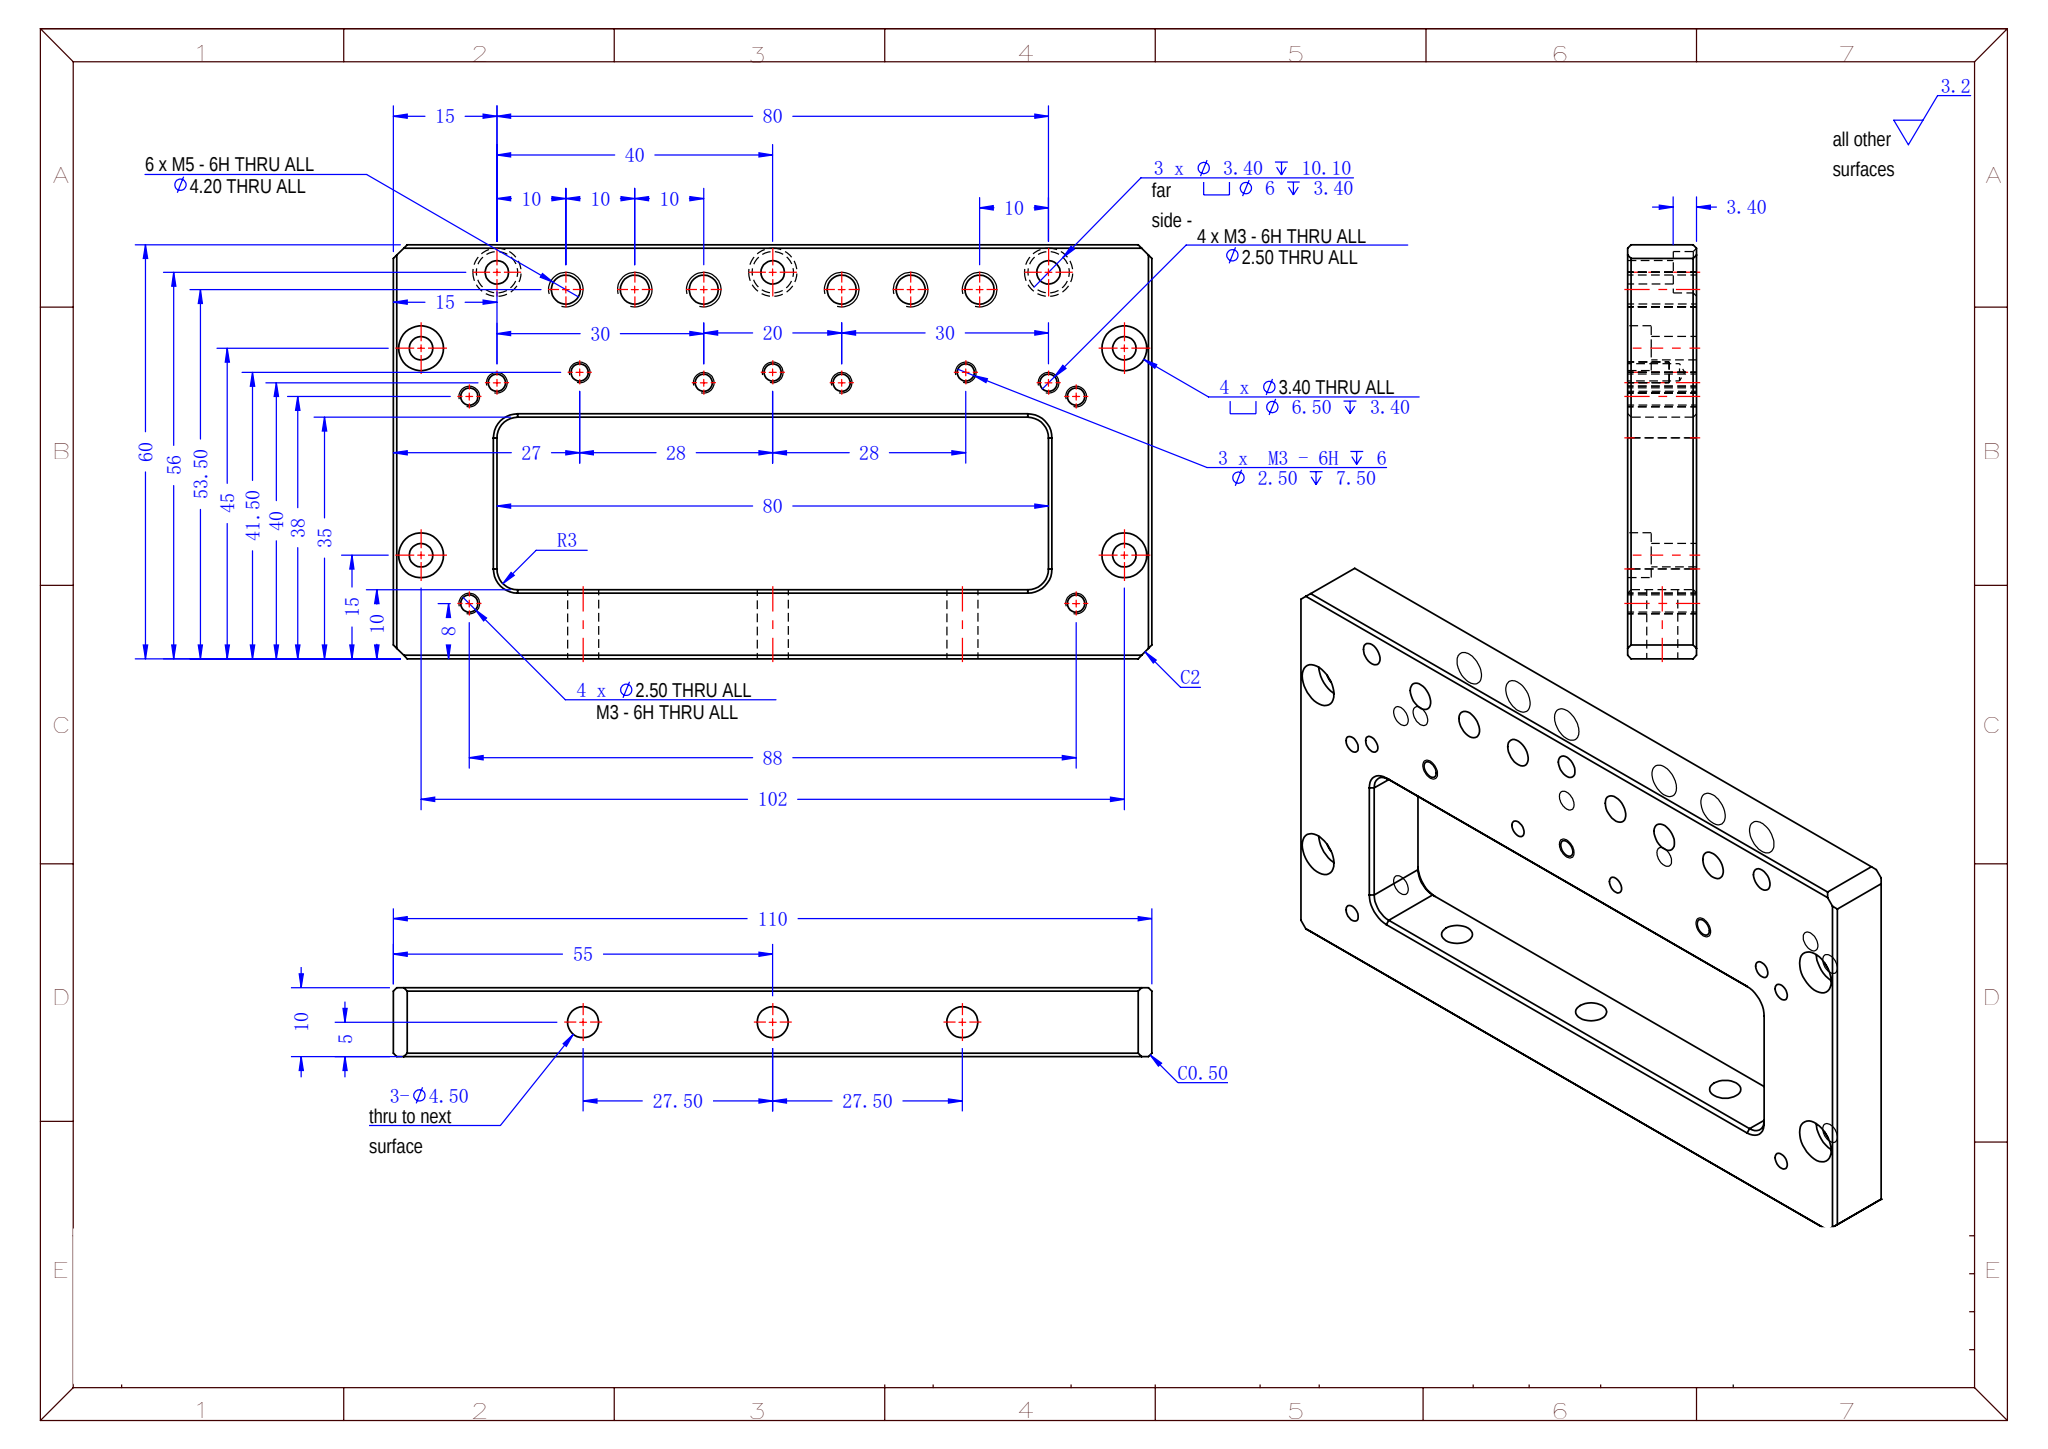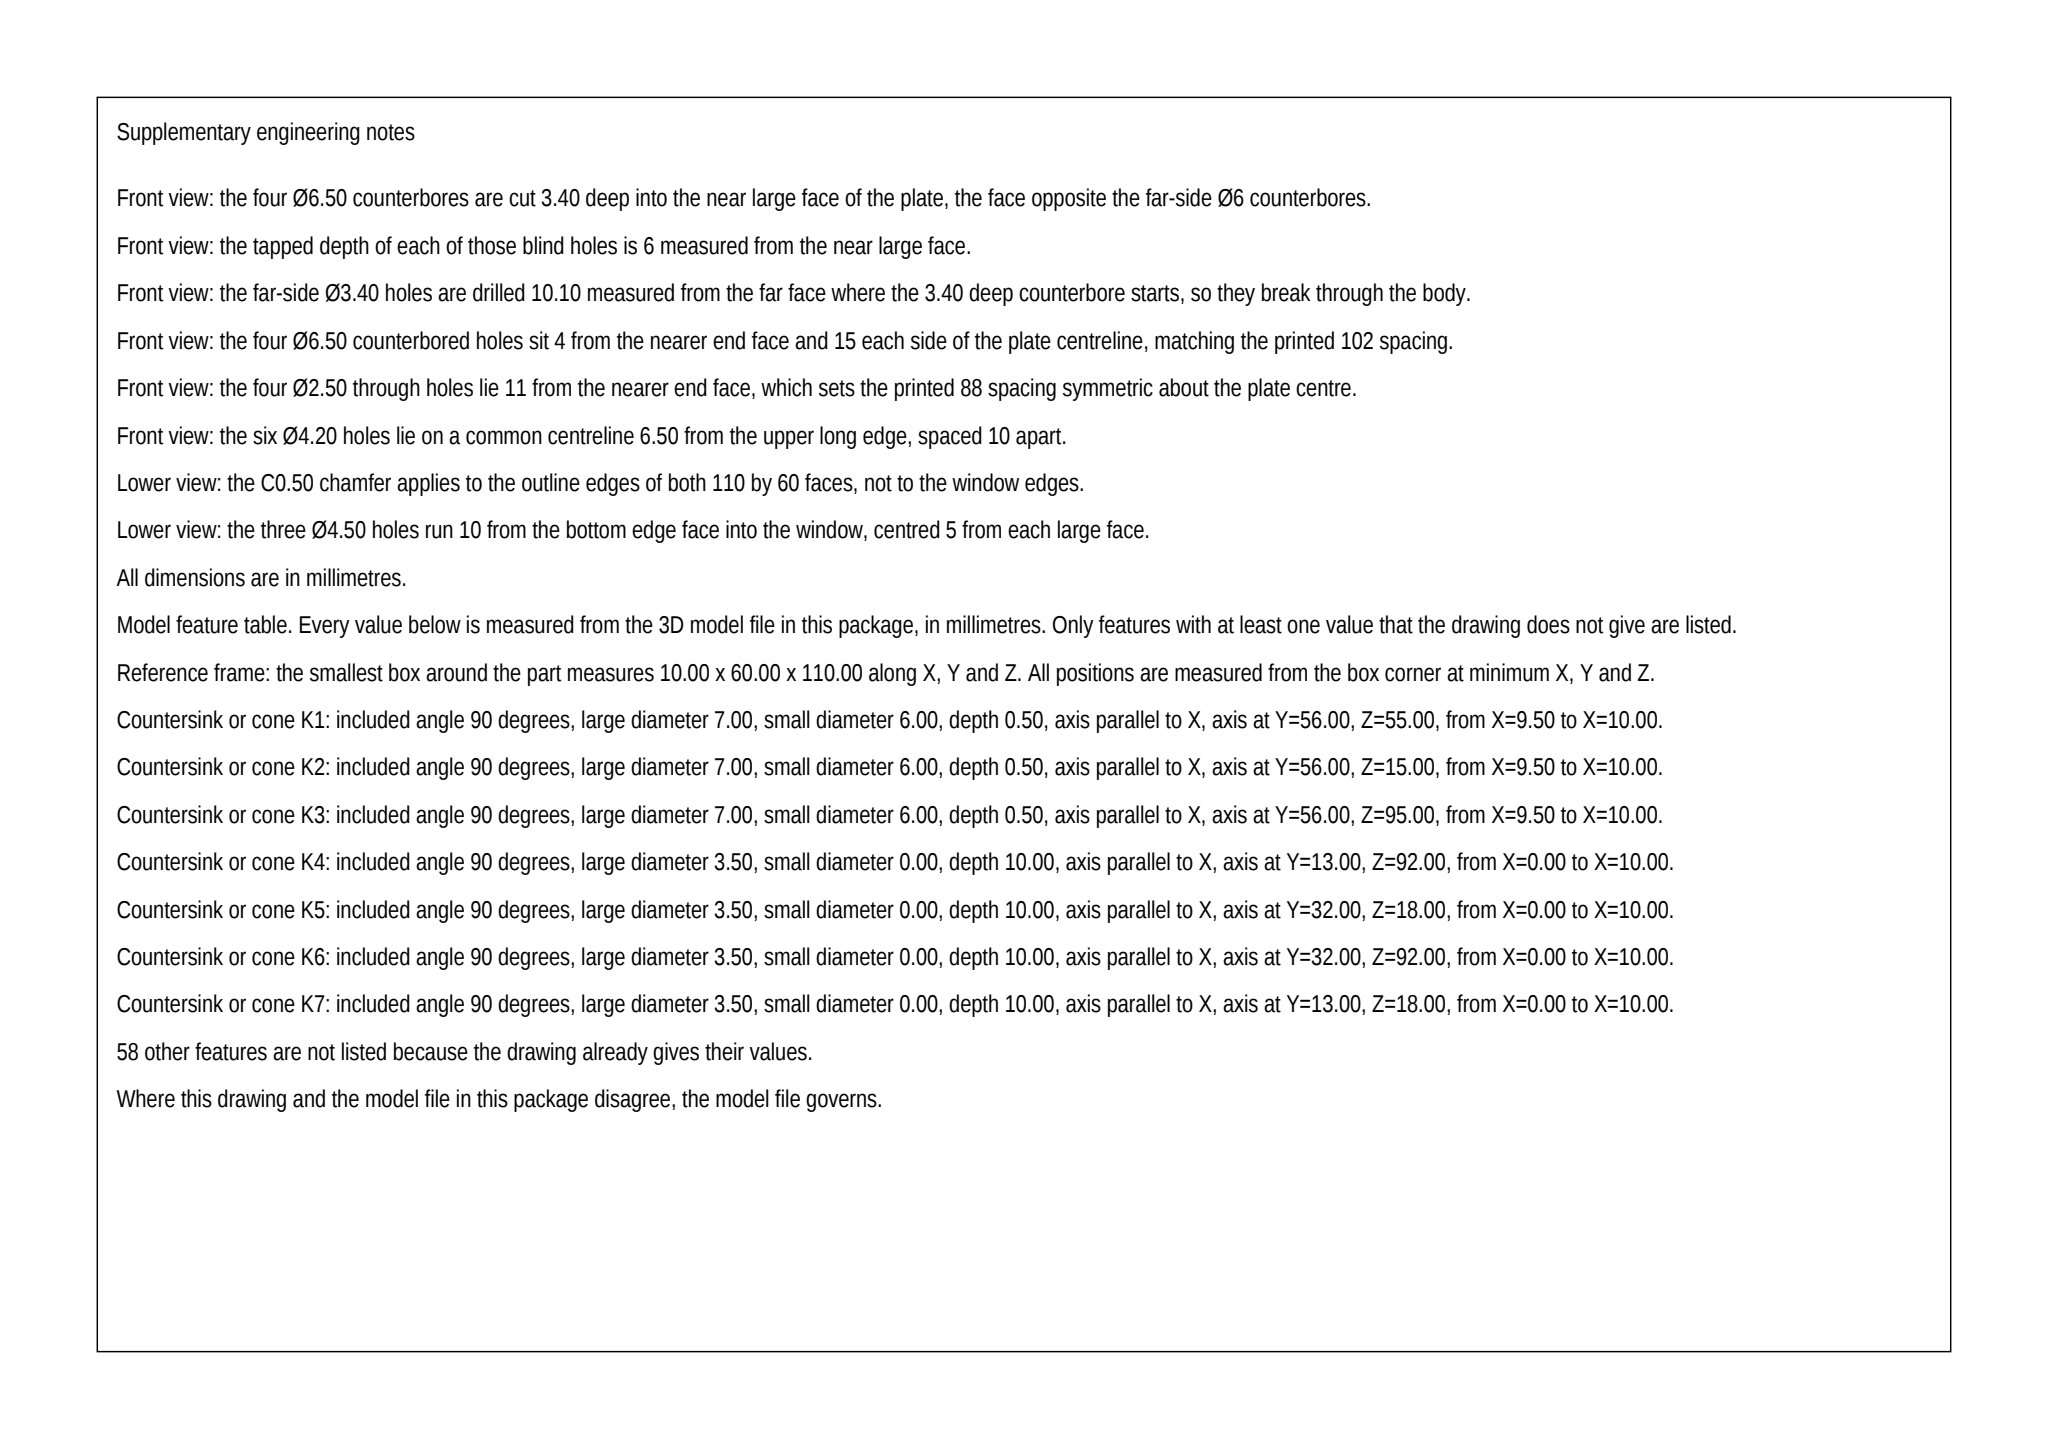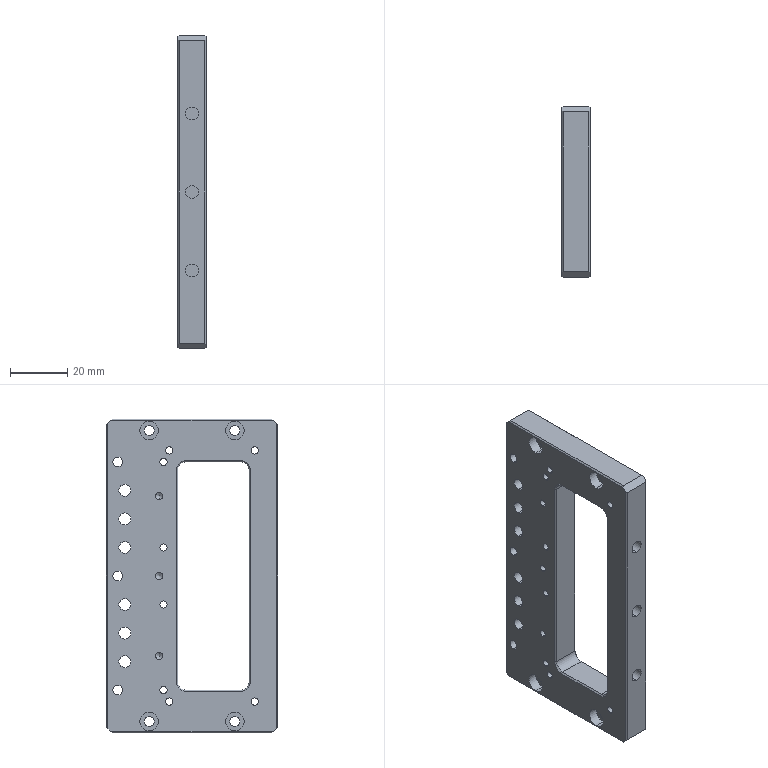Part | SolidWorks | mm | 1 solid | 129 faces | box 10 x 60 x 110 mm | volume 42883 mm3 | cylinder 72 | plane 37 | cone 20 | commonest cylinder face diameters 2.5 x22 3.4 x14 4.2 x12 6 x10 6.5 x8 4.5 x6
Drawing notes:
RECT POCKET 80 x 25, R3, DP 9 (1 THK FLOOR REMAINS) | from the solid: Part thk 10 (x-planes 0..10); pocket floor plane leaves 1 mm, depth 9
3-Ø4.50 DP 10 IN BOTTOM EDGE FACE, 5 FROM FACE | from the solid: cylinders [4.5,"y",[5.0,null,27.5/55.0/82.5],10.0]
5TH M5 HOLE: 75 FROM LH EDGE (10 FROM M5 AT 65) | from the solid: Ø4.20 thru cyl at z=75, y=53.5 in 6x M5 row (z=25,35,45,65,75,85); z datum = LH edge z=0